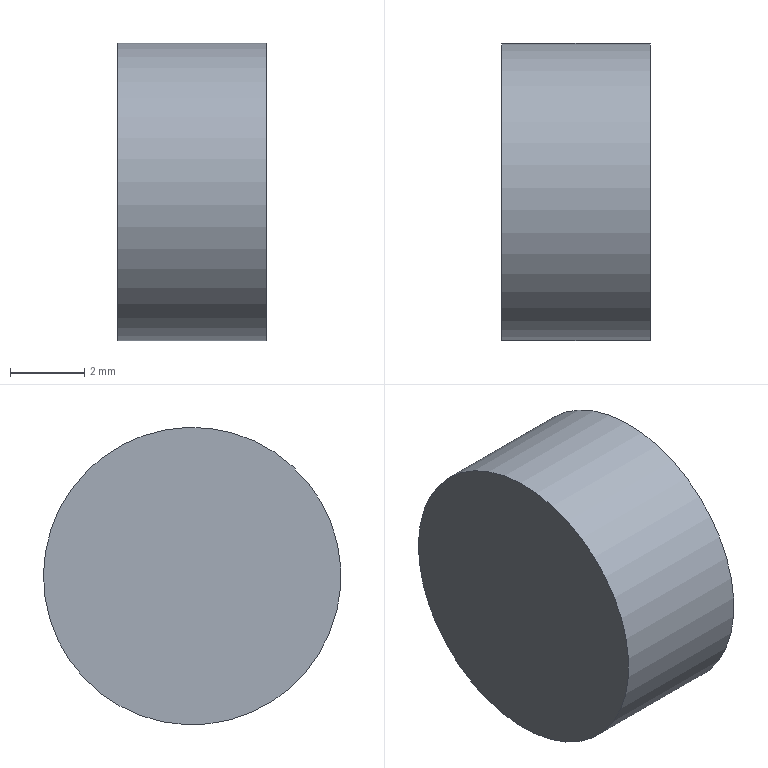Component | NX | BUTTON1 | 1 solid | 3 faces | box 4 x 8 x 8 mm | volume 201 mm3 | plane 2 | cylinder 1 | commonest cylinder face diameters 8 x1
STEP:
#1=CARTESIAN_POINT('',(0.,0.,0.));
#2=DIRECTION('',(0.,0.,1.));
#3=DIRECTION('',(1.,0.,0.));
#4=AXIS2_PLACEMENT_3D('',#1,#2,#3);
#5=CARTESIAN_POINT('',(-110.42,197.56,14.944));
#6=VERTEX_POINT('',#5);
#7=CARTESIAN_POINT('',(-110.42,201.257,16.472));
#8=DIRECTION('',(1.,0.,0.));
#9=DIRECTION('',(0.,-0.9242,-0.3818));
#10=AXIS2_PLACEMENT_3D('',#7,#8,#9);
#11=CIRCLE('',#10,4.);
#12=CARTESIAN_POINT('',(-110.42,201.257,16.472));
#13=DIRECTION('',(-1.,0.,0.));
#14=DIRECTION('',(0.,-0.9242,-0.3818));
#15=AXIS2_PLACEMENT_3D('',#12,#13,#14);
#16=PLANE('',#15);
#17=CARTESIAN_POINT('',(4.,0.));
#18=CARTESIAN_POINT('',(4.,-6.928));
#19=CARTESIAN_POINT('',(-2.,-3.464));
#20=CARTESIAN_POINT('',(-8.,-0.));
#21=CARTESIAN_POINT('',(-2.,3.464));
#22=CARTESIAN_POINT('',(4.,6.928));
#23=CARTESIAN_POINT('',(4.,0.));
#24=(BOUNDED_CURVE()B_SPLINE_CURVE(2,(#17,#18,#19,#20,#21,#22,#23),.UNSPECIFIED.,.T.,.F.)B_SPLINE_CURVE_WITH_KNOTS((1,2,2,2,2,1),(-2.094,0.,2.094,4.189,6.283,8.378),.UNSPECIFIED.)CURVE()GEOMETRIC_REPRESENTATION_ITEM()RATIONAL_B_SPLINE_CURVE((1.,0.5,1.,0.5,1.,0.5,1.))REPRESENTATION_ITEM(''));
#25=(GEOMETRIC_REPRESENTATION_CONTEXT(2)PARAMETRIC_REPRESENTATION_CONTEXT()REPRESENTATION_CONTEXT('',''));
#26=DEFINITIONAL_REPRESENTATION('',(#24),#25);
#27=PCURVE('',#16,#26);
#28=CARTESIAN_POINT('',(-106.42,201.257,16.472));
#29=DIRECTION('',(-1.,0.,0.));
#30=DIRECTION('',(0.,-0.9242,-0.3818));
#31=AXIS2_PLACEMENT_3D('',#28,#29,#30);
#32=CYLINDRICAL_SURFACE('',#31,4.);
#33=CARTESIAN_POINT('',(6.283,4.));
#34=DIRECTION('',(-1.,0.));
#35=VECTOR('',#34,1.);
#36=LINE('',#33,#35);
#37=(GEOMETRIC_REPRESENTATION_CONTEXT(2)PARAMETRIC_REPRESENTATION_CONTEXT()REPRESENTATION_CONTEXT('',''));
#38=DEFINITIONAL_REPRESENTATION('',(#36),#37);
#39=PCURVE('',#32,#38);
#40=SURFACE_CURVE('',#11,(#27,#39),.PCURVE_S1.);
#41=EDGE_CURVE('',#6,#6,#40,.T.);
#42=ORIENTED_EDGE('',*,*,#41,.F.);
#43=EDGE_LOOP('',(#42));
#44=FACE_BOUND('',#43,.T.);
#45=ADVANCED_FACE('',(#44),#16,.T.);
#46=CARTESIAN_POINT('',(-106.42,197.56,14.944));
#47=VERTEX_POINT('',#46);
#48=CARTESIAN_POINT('',(-106.42,201.257,16.472));
#49=DIRECTION('',(-1.,0.,0.));
#50=DIRECTION('',(0.,-0.9242,-0.3818));
#51=AXIS2_PLACEMENT_3D('',#48,#49,#50);
#52=CIRCLE('',#51,4.);
#53=CARTESIAN_POINT('',(-106.42,201.257,16.472));
#54=DIRECTION('',(1.,0.,0.));
#55=DIRECTION('',(0.,0.9242,0.3818));
#56=AXIS2_PLACEMENT_3D('',#53,#54,#55);
#57=PLANE('',#56);
#58=CARTESIAN_POINT('',(-4.,0.));
#59=CARTESIAN_POINT('',(-4.,6.928));
#60=CARTESIAN_POINT('',(2.,3.464));
#61=CARTESIAN_POINT('',(8.,-0.));
#62=CARTESIAN_POINT('',(2.,-3.464));
#63=CARTESIAN_POINT('',(-4.,-6.928));
#64=CARTESIAN_POINT('',(-4.,0.));
#65=(BOUNDED_CURVE()B_SPLINE_CURVE(2,(#58,#59,#60,#61,#62,#63,#64),.UNSPECIFIED.,.T.,.F.)B_SPLINE_CURVE_WITH_KNOTS((1,2,2,2,2,1),(-2.094,0.,2.094,4.189,6.283,8.378),.UNSPECIFIED.)CURVE()GEOMETRIC_REPRESENTATION_ITEM()RATIONAL_B_SPLINE_CURVE((1.,0.5,1.,0.5,1.,0.5,1.))REPRESENTATION_ITEM(''));
#66=(GEOMETRIC_REPRESENTATION_CONTEXT(2)PARAMETRIC_REPRESENTATION_CONTEXT()REPRESENTATION_CONTEXT('',''));
#67=DEFINITIONAL_REPRESENTATION('',(#65),#66);
#68=PCURVE('',#57,#67);
#69=CARTESIAN_POINT('',(0.,0.));
#70=DIRECTION('',(1.,0.));
#71=VECTOR('',#70,1.);
#72=LINE('',#69,#71);
#73=(GEOMETRIC_REPRESENTATION_CONTEXT(2)PARAMETRIC_REPRESENTATION_CONTEXT()REPRESENTATION_CONTEXT('',''));
#74=DEFINITIONAL_REPRESENTATION('',(#72),#73);
#75=PCURVE('',#32,#74);
#76=SURFACE_CURVE('',#52,(#68,#75),.PCURVE_S1.);
#77=EDGE_CURVE('',#47,#47,#76,.T.);
#78=ORIENTED_EDGE('',*,*,#77,.F.);
#79=EDGE_LOOP('',(#78));
#80=FACE_BOUND('',#79,.T.);
#81=ADVANCED_FACE('',(#80),#57,.T.);
#82=ORIENTED_EDGE('',*,*,#41,.T.);
#83=CARTESIAN_POINT('',(-106.42,197.56,14.944));
#84=CARTESIAN_POINT('',(-110.42,197.56,14.944));
#85=B_SPLINE_CURVE_WITH_KNOTS('',1,(#83,#84),.UNSPECIFIED.,.F.,.F.,(2,2),(0.,4.),.PIECEWISE_BEZIER_KNOTS.);
#86=CARTESIAN_POINT('',(0.,0.));
#87=DIRECTION('',(0.,1.));
#88=VECTOR('',#87,1.);
#89=LINE('',#86,#88);
#90=(GEOMETRIC_REPRESENTATION_CONTEXT(2)PARAMETRIC_REPRESENTATION_CONTEXT()REPRESENTATION_CONTEXT('',''));
#91=DEFINITIONAL_REPRESENTATION('',(#89),#90);
#92=PCURVE('',#32,#91);
#93=CARTESIAN_POINT('',(6.283,0.));
#94=DIRECTION('',(0.,1.));
#95=VECTOR('',#94,1.);
#96=LINE('',#93,#95);
#97=(GEOMETRIC_REPRESENTATION_CONTEXT(2)PARAMETRIC_REPRESENTATION_CONTEXT()REPRESENTATION_CONTEXT('',''));
#98=DEFINITIONAL_REPRESENTATION('',(#96),#97);
#99=PCURVE('',#32,#98);
#100=SEAM_CURVE('',#85,(#92,#99),.PCURVE_S1.);
#101=EDGE_CURVE('',#47,#6,#100,.T.);
#102=ORIENTED_EDGE('',*,*,#101,.F.);
#103=ORIENTED_EDGE('',*,*,#77,.T.);
#104=ORIENTED_EDGE('',*,*,#101,.T.);
#105=EDGE_LOOP('',(#82,#102,#103,#104));
#106=FACE_BOUND('',#105,.T.);
#107=ADVANCED_FACE('',(#106),#32,.T.);
#108=CLOSED_SHELL('',(#45,#81,#107));
#109=MANIFOLD_SOLID_BREP('',#108);
#110=(LENGTH_UNIT()NAMED_UNIT(*)SI_UNIT(.MILLI.,.METRE.));
#111=UNCERTAINTY_MEASURE_WITH_UNIT(LENGTH_MEASURE(0.00001),#110,'','');
#112=(NAMED_UNIT(*)PLANE_ANGLE_UNIT()SI_UNIT($,.RADIAN.));
#113=(NAMED_UNIT(*)SI_UNIT($,.STERADIAN.)SOLID_ANGLE_UNIT());
#114=(GEOMETRIC_REPRESENTATION_CONTEXT(3)GLOBAL_UNCERTAINTY_ASSIGNED_CONTEXT((#111))GLOBAL_UNIT_ASSIGNED_CONTEXT((#110,#112,#113))REPRESENTATION_CONTEXT('',''));
#115=ADVANCED_BREP_SHAPE_REPRESENTATION('',(#4,#109),#114);